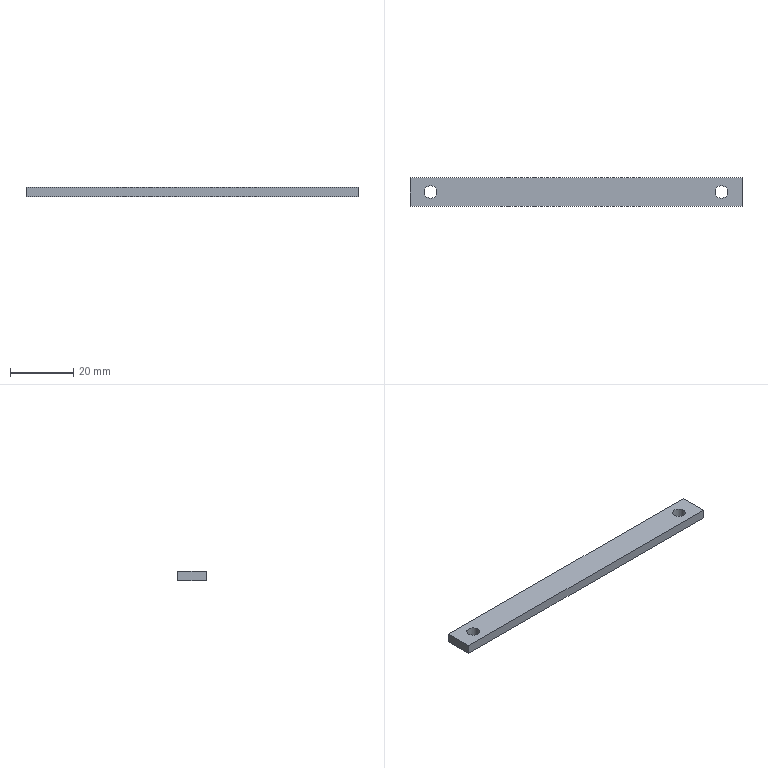Component | NX | GUIDE_PLATE_2 | 1 solid | 8 faces | box 105 x 9 x 3 mm | volume 2760 mm3 | plane 6 | cylinder 2 | commonest cylinder face diameters 4 x2
STEP:
#1=CARTESIAN_POINT('',(0.,0.,0.));
#2=DIRECTION('',(0.,0.,1.));
#3=DIRECTION('',(1.,0.,0.));
#4=AXIS2_PLACEMENT_3D('',#1,#2,#3);
#5=CARTESIAN_POINT('',(331.,-76.,115.5));
#6=VERTEX_POINT('',#5);
#7=CARTESIAN_POINT('',(226.,-76.,115.5));
#8=VERTEX_POINT('',#7);
#9=CARTESIAN_POINT('',(331.,-76.,115.5));
#10=DIRECTION('',(-1.,0.,0.));
#11=VECTOR('',#10,1.);
#12=LINE('',#9,#11);
#13=CARTESIAN_POINT('',(331.,-76.,118.5));
#14=DIRECTION('',(0.,-1.,0.));
#15=DIRECTION('',(0.,0.,-1.));
#16=AXIS2_PLACEMENT_3D('',#13,#14,#15);
#17=PLANE('',#16);
#18=CARTESIAN_POINT('',(3.,0.));
#19=DIRECTION('',(0.,-1.));
#20=VECTOR('',#19,1.);
#21=LINE('',#18,#20);
#22=(GEOMETRIC_REPRESENTATION_CONTEXT(2)PARAMETRIC_REPRESENTATION_CONTEXT()REPRESENTATION_CONTEXT('',''));
#23=DEFINITIONAL_REPRESENTATION('',(#21),#22);
#24=PCURVE('',#17,#23);
#25=CARTESIAN_POINT('',(324.5,-71.5,115.5));
#26=DIRECTION('',(0.,0.,1.));
#27=DIRECTION('',(1.,0.,0.));
#28=AXIS2_PLACEMENT_3D('',#25,#26,#27);
#29=PLANE('',#28);
#30=CARTESIAN_POINT('',(6.5,-4.5));
#31=DIRECTION('',(-1.,0.));
#32=VECTOR('',#31,1.);
#33=LINE('',#30,#32);
#34=(GEOMETRIC_REPRESENTATION_CONTEXT(2)PARAMETRIC_REPRESENTATION_CONTEXT()REPRESENTATION_CONTEXT('',''));
#35=DEFINITIONAL_REPRESENTATION('',(#33),#34);
#36=PCURVE('',#29,#35);
#37=SURFACE_CURVE('',#12,(#24,#36),.PCURVE_S1.);
#38=EDGE_CURVE('',#6,#8,#37,.T.);
#39=ORIENTED_EDGE('',*,*,#38,.F.);
#40=CARTESIAN_POINT('',(331.,-76.,118.5));
#41=VERTEX_POINT('',#40);
#42=CARTESIAN_POINT('',(331.,-76.,118.5));
#43=DIRECTION('',(0.,0.,-1.));
#44=VECTOR('',#43,1.);
#45=LINE('',#42,#44);
#46=CARTESIAN_POINT('',(0.,0.));
#47=DIRECTION('',(1.,0.));
#48=VECTOR('',#47,1.);
#49=LINE('',#46,#48);
#50=(GEOMETRIC_REPRESENTATION_CONTEXT(2)PARAMETRIC_REPRESENTATION_CONTEXT()REPRESENTATION_CONTEXT('',''));
#51=DEFINITIONAL_REPRESENTATION('',(#49),#50);
#52=PCURVE('',#17,#51);
#53=CARTESIAN_POINT('',(331.,-67.,118.5));
#54=DIRECTION('',(1.,0.,0.));
#55=DIRECTION('',(0.,0.,-1.));
#56=AXIS2_PLACEMENT_3D('',#53,#54,#55);
#57=PLANE('',#56);
#58=CARTESIAN_POINT('',(0.,-9.));
#59=DIRECTION('',(1.,0.));
#60=VECTOR('',#59,1.);
#61=LINE('',#58,#60);
#62=(GEOMETRIC_REPRESENTATION_CONTEXT(2)PARAMETRIC_REPRESENTATION_CONTEXT()REPRESENTATION_CONTEXT('',''));
#63=DEFINITIONAL_REPRESENTATION('',(#61),#62);
#64=PCURVE('',#57,#63);
#65=SURFACE_CURVE('',#45,(#52,#64),.PCURVE_S1.);
#66=EDGE_CURVE('',#41,#6,#65,.T.);
#67=ORIENTED_EDGE('',*,*,#66,.F.);
#68=CARTESIAN_POINT('',(226.,-76.,118.5));
#69=VERTEX_POINT('',#68);
#70=CARTESIAN_POINT('',(331.,-76.,118.5));
#71=DIRECTION('',(-1.,0.,0.));
#72=VECTOR('',#71,1.);
#73=LINE('',#70,#72);
#74=CARTESIAN_POINT('',(0.,0.));
#75=DIRECTION('',(0.,-1.));
#76=VECTOR('',#75,1.);
#77=LINE('',#74,#76);
#78=(GEOMETRIC_REPRESENTATION_CONTEXT(2)PARAMETRIC_REPRESENTATION_CONTEXT()REPRESENTATION_CONTEXT('',''));
#79=DEFINITIONAL_REPRESENTATION('',(#77),#78);
#80=PCURVE('',#17,#79);
#81=CARTESIAN_POINT('',(324.5,-71.5,118.5));
#82=DIRECTION('',(0.,0.,1.));
#83=DIRECTION('',(1.,0.,0.));
#84=AXIS2_PLACEMENT_3D('',#81,#82,#83);
#85=PLANE('',#84);
#86=CARTESIAN_POINT('',(6.5,-4.5));
#87=DIRECTION('',(-1.,0.));
#88=VECTOR('',#87,1.);
#89=LINE('',#86,#88);
#90=(GEOMETRIC_REPRESENTATION_CONTEXT(2)PARAMETRIC_REPRESENTATION_CONTEXT()REPRESENTATION_CONTEXT('',''));
#91=DEFINITIONAL_REPRESENTATION('',(#89),#90);
#92=PCURVE('',#85,#91);
#93=SURFACE_CURVE('',#73,(#80,#92),.PCURVE_S1.);
#94=EDGE_CURVE('',#41,#69,#93,.T.);
#95=ORIENTED_EDGE('',*,*,#94,.T.);
#96=CARTESIAN_POINT('',(226.,-76.,118.5));
#97=DIRECTION('',(0.,0.,-1.));
#98=VECTOR('',#97,1.);
#99=LINE('',#96,#98);
#100=CARTESIAN_POINT('',(0.,-105.));
#101=DIRECTION('',(1.,0.));
#102=VECTOR('',#101,1.);
#103=LINE('',#100,#102);
#104=(GEOMETRIC_REPRESENTATION_CONTEXT(2)PARAMETRIC_REPRESENTATION_CONTEXT()REPRESENTATION_CONTEXT('',''));
#105=DEFINITIONAL_REPRESENTATION('',(#103),#104);
#106=PCURVE('',#17,#105);
#107=CARTESIAN_POINT('',(226.,-76.,118.5));
#108=DIRECTION('',(-1.,0.,0.));
#109=DIRECTION('',(0.,0.,1.));
#110=AXIS2_PLACEMENT_3D('',#107,#108,#109);
#111=PLANE('',#110);
#112=CARTESIAN_POINT('',(0.,0.));
#113=DIRECTION('',(-1.,0.));
#114=VECTOR('',#113,1.);
#115=LINE('',#112,#114);
#116=(GEOMETRIC_REPRESENTATION_CONTEXT(2)PARAMETRIC_REPRESENTATION_CONTEXT()REPRESENTATION_CONTEXT('',''));
#117=DEFINITIONAL_REPRESENTATION('',(#115),#116);
#118=PCURVE('',#111,#117);
#119=SURFACE_CURVE('',#99,(#106,#118),.PCURVE_S1.);
#120=EDGE_CURVE('',#69,#8,#119,.T.);
#121=ORIENTED_EDGE('',*,*,#120,.T.);
#122=EDGE_LOOP('',(#39,#67,#95,#121));
#123=FACE_BOUND('',#122,.T.);
#124=ADVANCED_FACE('',(#123),#17,.T.);
#125=CARTESIAN_POINT('',(226.,-67.,115.5));
#126=VERTEX_POINT('',#125);
#127=CARTESIAN_POINT('',(226.,-76.,115.5));
#128=DIRECTION('',(0.,1.,0.));
#129=VECTOR('',#128,1.);
#130=LINE('',#127,#129);
#131=CARTESIAN_POINT('',(-3.,0.));
#132=DIRECTION('',(0.,1.));
#133=VECTOR('',#132,1.);
#134=LINE('',#131,#133);
#135=(GEOMETRIC_REPRESENTATION_CONTEXT(2)PARAMETRIC_REPRESENTATION_CONTEXT()REPRESENTATION_CONTEXT('',''));
#136=DEFINITIONAL_REPRESENTATION('',(#134),#135);
#137=PCURVE('',#111,#136);
#138=CARTESIAN_POINT('',(-98.5,-4.5));
#139=DIRECTION('',(0.,1.));
#140=VECTOR('',#139,1.);
#141=LINE('',#138,#140);
#142=(GEOMETRIC_REPRESENTATION_CONTEXT(2)PARAMETRIC_REPRESENTATION_CONTEXT()REPRESENTATION_CONTEXT('',''));
#143=DEFINITIONAL_REPRESENTATION('',(#141),#142);
#144=PCURVE('',#29,#143);
#145=SURFACE_CURVE('',#130,(#137,#144),.PCURVE_S1.);
#146=EDGE_CURVE('',#8,#126,#145,.T.);
#147=ORIENTED_EDGE('',*,*,#146,.F.);
#148=ORIENTED_EDGE('',*,*,#120,.F.);
#149=CARTESIAN_POINT('',(226.,-67.,118.5));
#150=VERTEX_POINT('',#149);
#151=CARTESIAN_POINT('',(226.,-76.,118.5));
#152=DIRECTION('',(0.,1.,0.));
#153=VECTOR('',#152,1.);
#154=LINE('',#151,#153);
#155=CARTESIAN_POINT('',(0.,0.));
#156=DIRECTION('',(0.,1.));
#157=VECTOR('',#156,1.);
#158=LINE('',#155,#157);
#159=(GEOMETRIC_REPRESENTATION_CONTEXT(2)PARAMETRIC_REPRESENTATION_CONTEXT()REPRESENTATION_CONTEXT('',''));
#160=DEFINITIONAL_REPRESENTATION('',(#158),#159);
#161=PCURVE('',#111,#160);
#162=CARTESIAN_POINT('',(-98.5,-4.5));
#163=DIRECTION('',(0.,1.));
#164=VECTOR('',#163,1.);
#165=LINE('',#162,#164);
#166=(GEOMETRIC_REPRESENTATION_CONTEXT(2)PARAMETRIC_REPRESENTATION_CONTEXT()REPRESENTATION_CONTEXT('',''));
#167=DEFINITIONAL_REPRESENTATION('',(#165),#166);
#168=PCURVE('',#85,#167);
#169=SURFACE_CURVE('',#154,(#161,#168),.PCURVE_S1.);
#170=EDGE_CURVE('',#69,#150,#169,.T.);
#171=ORIENTED_EDGE('',*,*,#170,.T.);
#172=CARTESIAN_POINT('',(226.,-67.,118.5));
#173=DIRECTION('',(0.,0.,-1.));
#174=VECTOR('',#173,1.);
#175=LINE('',#172,#174);
#176=CARTESIAN_POINT('',(0.,9.));
#177=DIRECTION('',(-1.,0.));
#178=VECTOR('',#177,1.);
#179=LINE('',#176,#178);
#180=(GEOMETRIC_REPRESENTATION_CONTEXT(2)PARAMETRIC_REPRESENTATION_CONTEXT()REPRESENTATION_CONTEXT('',''));
#181=DEFINITIONAL_REPRESENTATION('',(#179),#180);
#182=PCURVE('',#111,#181);
#183=CARTESIAN_POINT('',(226.,-67.,118.5));
#184=DIRECTION('',(0.,1.,0.));
#185=DIRECTION('',(0.,0.,1.));
#186=AXIS2_PLACEMENT_3D('',#183,#184,#185);
#187=PLANE('',#186);
#188=CARTESIAN_POINT('',(0.,0.));
#189=DIRECTION('',(-1.,0.));
#190=VECTOR('',#189,1.);
#191=LINE('',#188,#190);
#192=(GEOMETRIC_REPRESENTATION_CONTEXT(2)PARAMETRIC_REPRESENTATION_CONTEXT()REPRESENTATION_CONTEXT('',''));
#193=DEFINITIONAL_REPRESENTATION('',(#191),#192);
#194=PCURVE('',#187,#193);
#195=SURFACE_CURVE('',#175,(#182,#194),.PCURVE_S1.);
#196=EDGE_CURVE('',#150,#126,#195,.T.);
#197=ORIENTED_EDGE('',*,*,#196,.T.);
#198=EDGE_LOOP('',(#147,#148,#171,#197));
#199=FACE_BOUND('',#198,.T.);
#200=ADVANCED_FACE('',(#199),#111,.T.);
#201=CARTESIAN_POINT('',(331.,-67.,115.5));
#202=VERTEX_POINT('',#201);
#203=CARTESIAN_POINT('',(226.,-67.,115.5));
#204=DIRECTION('',(1.,0.,0.));
#205=VECTOR('',#204,1.);
#206=LINE('',#203,#205);
#207=CARTESIAN_POINT('',(-3.,0.));
#208=DIRECTION('',(0.,1.));
#209=VECTOR('',#208,1.);
#210=LINE('',#207,#209);
#211=(GEOMETRIC_REPRESENTATION_CONTEXT(2)PARAMETRIC_REPRESENTATION_CONTEXT()REPRESENTATION_CONTEXT('',''));
#212=DEFINITIONAL_REPRESENTATION('',(#210),#211);
#213=PCURVE('',#187,#212);
#214=CARTESIAN_POINT('',(-98.5,4.5));
#215=DIRECTION('',(1.,0.));
#216=VECTOR('',#215,1.);
#217=LINE('',#214,#216);
#218=(GEOMETRIC_REPRESENTATION_CONTEXT(2)PARAMETRIC_REPRESENTATION_CONTEXT()REPRESENTATION_CONTEXT('',''));
#219=DEFINITIONAL_REPRESENTATION('',(#217),#218);
#220=PCURVE('',#29,#219);
#221=SURFACE_CURVE('',#206,(#213,#220),.PCURVE_S1.);
#222=EDGE_CURVE('',#126,#202,#221,.T.);
#223=ORIENTED_EDGE('',*,*,#222,.F.);
#224=ORIENTED_EDGE('',*,*,#196,.F.);
#225=CARTESIAN_POINT('',(331.,-67.,118.5));
#226=VERTEX_POINT('',#225);
#227=CARTESIAN_POINT('',(226.,-67.,118.5));
#228=DIRECTION('',(1.,0.,0.));
#229=VECTOR('',#228,1.);
#230=LINE('',#227,#229);
#231=CARTESIAN_POINT('',(0.,0.));
#232=DIRECTION('',(0.,1.));
#233=VECTOR('',#232,1.);
#234=LINE('',#231,#233);
#235=(GEOMETRIC_REPRESENTATION_CONTEXT(2)PARAMETRIC_REPRESENTATION_CONTEXT()REPRESENTATION_CONTEXT('',''));
#236=DEFINITIONAL_REPRESENTATION('',(#234),#235);
#237=PCURVE('',#187,#236);
#238=CARTESIAN_POINT('',(-98.5,4.5));
#239=DIRECTION('',(1.,0.));
#240=VECTOR('',#239,1.);
#241=LINE('',#238,#240);
#242=(GEOMETRIC_REPRESENTATION_CONTEXT(2)PARAMETRIC_REPRESENTATION_CONTEXT()REPRESENTATION_CONTEXT('',''));
#243=DEFINITIONAL_REPRESENTATION('',(#241),#242);
#244=PCURVE('',#85,#243);
#245=SURFACE_CURVE('',#230,(#237,#244),.PCURVE_S1.);
#246=EDGE_CURVE('',#150,#226,#245,.T.);
#247=ORIENTED_EDGE('',*,*,#246,.T.);
#248=CARTESIAN_POINT('',(331.,-67.,118.5));
#249=DIRECTION('',(0.,0.,-1.));
#250=VECTOR('',#249,1.);
#251=LINE('',#248,#250);
#252=CARTESIAN_POINT('',(0.,105.));
#253=DIRECTION('',(-1.,0.));
#254=VECTOR('',#253,1.);
#255=LINE('',#252,#254);
#256=(GEOMETRIC_REPRESENTATION_CONTEXT(2)PARAMETRIC_REPRESENTATION_CONTEXT()REPRESENTATION_CONTEXT('',''));
#257=DEFINITIONAL_REPRESENTATION('',(#255),#256);
#258=PCURVE('',#187,#257);
#259=CARTESIAN_POINT('',(0.,0.));
#260=DIRECTION('',(1.,0.));
#261=VECTOR('',#260,1.);
#262=LINE('',#259,#261);
#263=(GEOMETRIC_REPRESENTATION_CONTEXT(2)PARAMETRIC_REPRESENTATION_CONTEXT()REPRESENTATION_CONTEXT('',''));
#264=DEFINITIONAL_REPRESENTATION('',(#262),#263);
#265=PCURVE('',#57,#264);
#266=SURFACE_CURVE('',#251,(#258,#265),.PCURVE_S1.);
#267=EDGE_CURVE('',#226,#202,#266,.T.);
#268=ORIENTED_EDGE('',*,*,#267,.T.);
#269=EDGE_LOOP('',(#223,#224,#247,#268));
#270=FACE_BOUND('',#269,.T.);
#271=ADVANCED_FACE('',(#270),#187,.T.);
#272=CARTESIAN_POINT('',(322.5,-71.5,118.5));
#273=VERTEX_POINT('',#272);
#274=CARTESIAN_POINT('',(324.5,-71.5,118.5));
#275=DIRECTION('',(0.,0.,1.));
#276=DIRECTION('',(-1.,0.,0.));
#277=AXIS2_PLACEMENT_3D('',#274,#275,#276);
#278=CIRCLE('',#277,2.);
#279=CARTESIAN_POINT('',(324.5,-71.5,118.5));
#280=DIRECTION('',(0.,0.,-1.));
#281=DIRECTION('',(-1.,0.,0.));
#282=AXIS2_PLACEMENT_3D('',#279,#280,#281);
#283=CYLINDRICAL_SURFACE('',#282,2.);
#284=CARTESIAN_POINT('',(6.283,0.));
#285=DIRECTION('',(-1.,0.));
#286=VECTOR('',#285,1.);
#287=LINE('',#284,#286);
#288=(GEOMETRIC_REPRESENTATION_CONTEXT(2)PARAMETRIC_REPRESENTATION_CONTEXT()REPRESENTATION_CONTEXT('',''));
#289=DEFINITIONAL_REPRESENTATION('',(#287),#288);
#290=PCURVE('',#283,#289);
#291=CARTESIAN_POINT('',(0.,0.));
#292=DIRECTION('',(-1.,0.));
#293=AXIS2_PLACEMENT_2D('',#291,#292);
#294=CIRCLE('',#293,2.);
#295=(GEOMETRIC_REPRESENTATION_CONTEXT(2)PARAMETRIC_REPRESENTATION_CONTEXT()REPRESENTATION_CONTEXT('',''));
#296=DEFINITIONAL_REPRESENTATION('',(#294),#295);
#297=PCURVE('',#85,#296);
#298=SURFACE_CURVE('',#278,(#290,#297),.PCURVE_S1.);
#299=EDGE_CURVE('',#273,#273,#298,.T.);
#300=ORIENTED_EDGE('',*,*,#299,.F.);
#301=CARTESIAN_POINT('',(322.5,-71.5,115.5));
#302=VERTEX_POINT('',#301);
#303=CARTESIAN_POINT('',(322.5,-71.5,118.5));
#304=CARTESIAN_POINT('',(322.5,-71.5,115.5));
#305=B_SPLINE_CURVE_WITH_KNOTS('',1,(#303,#304),.UNSPECIFIED.,.F.,.F.,(2,2),(0.,3.),.PIECEWISE_BEZIER_KNOTS.);
#306=CARTESIAN_POINT('',(6.283,0.));
#307=DIRECTION('',(0.,1.));
#308=VECTOR('',#307,1.);
#309=LINE('',#306,#308);
#310=(GEOMETRIC_REPRESENTATION_CONTEXT(2)PARAMETRIC_REPRESENTATION_CONTEXT()REPRESENTATION_CONTEXT('',''));
#311=DEFINITIONAL_REPRESENTATION('',(#309),#310);
#312=PCURVE('',#283,#311);
#313=CARTESIAN_POINT('',(0.,0.));
#314=DIRECTION('',(0.,1.));
#315=VECTOR('',#314,1.);
#316=LINE('',#313,#315);
#317=(GEOMETRIC_REPRESENTATION_CONTEXT(2)PARAMETRIC_REPRESENTATION_CONTEXT()REPRESENTATION_CONTEXT('',''));
#318=DEFINITIONAL_REPRESENTATION('',(#316),#317);
#319=PCURVE('',#283,#318);
#320=SEAM_CURVE('',#305,(#312,#319),.PCURVE_S1.);
#321=EDGE_CURVE('',#273,#302,#320,.T.);
#322=ORIENTED_EDGE('',*,*,#321,.T.);
#323=CARTESIAN_POINT('',(324.5,-71.5,115.5));
#324=DIRECTION('',(0.,0.,1.));
#325=DIRECTION('',(-1.,0.,0.));
#326=AXIS2_PLACEMENT_3D('',#323,#324,#325);
#327=CIRCLE('',#326,2.);
#328=CARTESIAN_POINT('',(6.283,3.));
#329=DIRECTION('',(-1.,0.));
#330=VECTOR('',#329,1.);
#331=LINE('',#328,#330);
#332=(GEOMETRIC_REPRESENTATION_CONTEXT(2)PARAMETRIC_REPRESENTATION_CONTEXT()REPRESENTATION_CONTEXT('',''));
#333=DEFINITIONAL_REPRESENTATION('',(#331),#332);
#334=PCURVE('',#283,#333);
#335=CARTESIAN_POINT('',(0.,0.));
#336=DIRECTION('',(-1.,0.));
#337=AXIS2_PLACEMENT_2D('',#335,#336);
#338=CIRCLE('',#337,2.);
#339=(GEOMETRIC_REPRESENTATION_CONTEXT(2)PARAMETRIC_REPRESENTATION_CONTEXT()REPRESENTATION_CONTEXT('',''));
#340=DEFINITIONAL_REPRESENTATION('',(#338),#339);
#341=PCURVE('',#29,#340);
#342=SURFACE_CURVE('',#327,(#334,#341),.PCURVE_S1.);
#343=EDGE_CURVE('',#302,#302,#342,.T.);
#344=ORIENTED_EDGE('',*,*,#343,.T.);
#345=ORIENTED_EDGE('',*,*,#321,.F.);
#346=EDGE_LOOP('',(#300,#322,#344,#345));
#347=FACE_BOUND('',#346,.F.);
#348=ADVANCED_FACE('',(#347),#283,.F.);
#349=CARTESIAN_POINT('',(331.,-67.,115.5));
#350=DIRECTION('',(0.,-1.,0.));
#351=VECTOR('',#350,1.);
#352=LINE('',#349,#351);
#353=CARTESIAN_POINT('',(3.,0.));
#354=DIRECTION('',(0.,-1.));
#355=VECTOR('',#354,1.);
#356=LINE('',#353,#355);
#357=(GEOMETRIC_REPRESENTATION_CONTEXT(2)PARAMETRIC_REPRESENTATION_CONTEXT()REPRESENTATION_CONTEXT('',''));
#358=DEFINITIONAL_REPRESENTATION('',(#356),#357);
#359=PCURVE('',#57,#358);
#360=CARTESIAN_POINT('',(6.5,4.5));
#361=DIRECTION('',(0.,-1.));
#362=VECTOR('',#361,1.);
#363=LINE('',#360,#362);
#364=(GEOMETRIC_REPRESENTATION_CONTEXT(2)PARAMETRIC_REPRESENTATION_CONTEXT()REPRESENTATION_CONTEXT('',''));
#365=DEFINITIONAL_REPRESENTATION('',(#363),#364);
#366=PCURVE('',#29,#365);
#367=SURFACE_CURVE('',#352,(#359,#366),.PCURVE_S1.);
#368=EDGE_CURVE('',#202,#6,#367,.T.);
#369=ORIENTED_EDGE('',*,*,#368,.F.);
#370=ORIENTED_EDGE('',*,*,#267,.F.);
#371=CARTESIAN_POINT('',(331.,-67.,118.5));
#372=DIRECTION('',(0.,-1.,0.));
#373=VECTOR('',#372,1.);
#374=LINE('',#371,#373);
#375=CARTESIAN_POINT('',(0.,0.));
#376=DIRECTION('',(0.,-1.));
#377=VECTOR('',#376,1.);
#378=LINE('',#375,#377);
#379=(GEOMETRIC_REPRESENTATION_CONTEXT(2)PARAMETRIC_REPRESENTATION_CONTEXT()REPRESENTATION_CONTEXT('',''));
#380=DEFINITIONAL_REPRESENTATION('',(#378),#379);
#381=PCURVE('',#57,#380);
#382=CARTESIAN_POINT('',(6.5,4.5));
#383=DIRECTION('',(0.,-1.));
#384=VECTOR('',#383,1.);
#385=LINE('',#382,#384);
#386=(GEOMETRIC_REPRESENTATION_CONTEXT(2)PARAMETRIC_REPRESENTATION_CONTEXT()REPRESENTATION_CONTEXT('',''));
#387=DEFINITIONAL_REPRESENTATION('',(#385),#386);
#388=PCURVE('',#85,#387);
#389=SURFACE_CURVE('',#374,(#381,#388),.PCURVE_S1.);
#390=EDGE_CURVE('',#226,#41,#389,.T.);
#391=ORIENTED_EDGE('',*,*,#390,.T.);
#392=ORIENTED_EDGE('',*,*,#66,.T.);
#393=EDGE_LOOP('',(#369,#370,#391,#392));
#394=FACE_BOUND('',#393,.T.);
#395=ADVANCED_FACE('',(#394),#57,.T.);
#396=CARTESIAN_POINT('',(234.5,-71.5,118.5));
#397=VERTEX_POINT('',#396);
#398=CARTESIAN_POINT('',(232.5,-71.5,118.5));
#399=DIRECTION('',(0.,0.,-1.));
#400=DIRECTION('',(1.,0.,0.));
#401=AXIS2_PLACEMENT_3D('',#398,#399,#400);
#402=CIRCLE('',#401,2.);
#403=CARTESIAN_POINT('',(232.5,-71.5,118.5));
#404=DIRECTION('',(0.,0.,-1.));
#405=DIRECTION('',(-1.,0.,0.));
#406=AXIS2_PLACEMENT_3D('',#403,#404,#405);
#407=CYLINDRICAL_SURFACE('',#406,2.);
#408=CARTESIAN_POINT('',(3.142,0.));
#409=DIRECTION('',(1.,0.));
#410=VECTOR('',#409,1.);
#411=LINE('',#408,#410);
#412=(GEOMETRIC_REPRESENTATION_CONTEXT(2)PARAMETRIC_REPRESENTATION_CONTEXT()REPRESENTATION_CONTEXT('',''));
#413=DEFINITIONAL_REPRESENTATION('',(#411),#412);
#414=PCURVE('',#407,#413);
#415=CARTESIAN_POINT('',(-90.,0.));
#416=CARTESIAN_POINT('',(-90.,-3.464));
#417=CARTESIAN_POINT('',(-93.,-1.732));
#418=CARTESIAN_POINT('',(-96.,-0.));
#419=CARTESIAN_POINT('',(-93.,1.732));
#420=CARTESIAN_POINT('',(-90.,3.464));
#421=CARTESIAN_POINT('',(-90.,0.));
#422=(BOUNDED_CURVE()B_SPLINE_CURVE(2,(#415,#416,#417,#418,#419,#420,#421),.UNSPECIFIED.,.T.,.F.)B_SPLINE_CURVE_WITH_KNOTS((1,2,2,2,2,1),(-2.094,0.,2.094,4.189,6.283,8.378),.UNSPECIFIED.)CURVE()GEOMETRIC_REPRESENTATION_ITEM()RATIONAL_B_SPLINE_CURVE((1.,0.5,1.,0.5,1.,0.5,1.))REPRESENTATION_ITEM(''));
#423=(GEOMETRIC_REPRESENTATION_CONTEXT(2)PARAMETRIC_REPRESENTATION_CONTEXT()REPRESENTATION_CONTEXT('',''));
#424=DEFINITIONAL_REPRESENTATION('',(#422),#423);
#425=PCURVE('',#85,#424);
#426=SURFACE_CURVE('',#402,(#414,#425),.PCURVE_S1.);
#427=EDGE_CURVE('',#397,#397,#426,.T.);
#428=ORIENTED_EDGE('',*,*,#427,.T.);
#429=CARTESIAN_POINT('',(234.5,-71.5,115.5));
#430=VERTEX_POINT('',#429);
#431=CARTESIAN_POINT('',(234.5,-71.5,118.5));
#432=CARTESIAN_POINT('',(234.5,-71.5,115.5));
#433=B_SPLINE_CURVE_WITH_KNOTS('',1,(#431,#432),.UNSPECIFIED.,.F.,.F.,(2,2),(0.,3.),.PIECEWISE_BEZIER_KNOTS.);
#434=CARTESIAN_POINT('',(9.425,0.));
#435=DIRECTION('',(0.,1.));
#436=VECTOR('',#435,1.);
#437=LINE('',#434,#436);
#438=(GEOMETRIC_REPRESENTATION_CONTEXT(2)PARAMETRIC_REPRESENTATION_CONTEXT()REPRESENTATION_CONTEXT('',''));
#439=DEFINITIONAL_REPRESENTATION('',(#437),#438);
#440=PCURVE('',#407,#439);
#441=CARTESIAN_POINT('',(3.142,0.));
#442=DIRECTION('',(0.,1.));
#443=VECTOR('',#442,1.);
#444=LINE('',#441,#443);
#445=(GEOMETRIC_REPRESENTATION_CONTEXT(2)PARAMETRIC_REPRESENTATION_CONTEXT()REPRESENTATION_CONTEXT('',''));
#446=DEFINITIONAL_REPRESENTATION('',(#444),#445);
#447=PCURVE('',#407,#446);
#448=SEAM_CURVE('',#433,(#440,#447),.PCURVE_S1.);
#449=EDGE_CURVE('',#397,#430,#448,.T.);
#450=ORIENTED_EDGE('',*,*,#449,.T.);
#451=CARTESIAN_POINT('',(232.5,-71.5,115.5));
#452=DIRECTION('',(0.,0.,-1.));
#453=DIRECTION('',(1.,0.,0.));
#454=AXIS2_PLACEMENT_3D('',#451,#452,#453);
#455=CIRCLE('',#454,2.);
#456=CARTESIAN_POINT('',(3.142,3.));
#457=DIRECTION('',(1.,0.));
#458=VECTOR('',#457,1.);
#459=LINE('',#456,#458);
#460=(GEOMETRIC_REPRESENTATION_CONTEXT(2)PARAMETRIC_REPRESENTATION_CONTEXT()REPRESENTATION_CONTEXT('',''));
#461=DEFINITIONAL_REPRESENTATION('',(#459),#460);
#462=PCURVE('',#407,#461);
#463=CARTESIAN_POINT('',(-90.,0.));
#464=CARTESIAN_POINT('',(-90.,-3.464));
#465=CARTESIAN_POINT('',(-93.,-1.732));
#466=CARTESIAN_POINT('',(-96.,-0.));
#467=CARTESIAN_POINT('',(-93.,1.732));
#468=CARTESIAN_POINT('',(-90.,3.464));
#469=CARTESIAN_POINT('',(-90.,0.));
#470=(BOUNDED_CURVE()B_SPLINE_CURVE(2,(#463,#464,#465,#466,#467,#468,#469),.UNSPECIFIED.,.T.,.F.)B_SPLINE_CURVE_WITH_KNOTS((1,2,2,2,2,1),(-2.094,0.,2.094,4.189,6.283,8.378),.UNSPECIFIED.)CURVE()GEOMETRIC_REPRESENTATION_ITEM()RATIONAL_B_SPLINE_CURVE((1.,0.5,1.,0.5,1.,0.5,1.))REPRESENTATION_ITEM(''));
#471=(GEOMETRIC_REPRESENTATION_CONTEXT(2)PARAMETRIC_REPRESENTATION_CONTEXT()REPRESENTATION_CONTEXT('',''));
#472=DEFINITIONAL_REPRESENTATION('',(#470),#471);
#473=PCURVE('',#29,#472);
#474=SURFACE_CURVE('',#455,(#462,#473),.PCURVE_S1.);
#475=EDGE_CURVE('',#430,#430,#474,.T.);
#476=ORIENTED_EDGE('',*,*,#475,.F.);
#477=ORIENTED_EDGE('',*,*,#449,.F.);
#478=EDGE_LOOP('',(#428,#450,#476,#477));
#479=FACE_BOUND('',#478,.F.);
#480=ADVANCED_FACE('',(#479),#407,.F.);
#481=ORIENTED_EDGE('',*,*,#94,.F.);
#482=ORIENTED_EDGE('',*,*,#390,.F.);
#483=ORIENTED_EDGE('',*,*,#246,.F.);
#484=ORIENTED_EDGE('',*,*,#170,.F.);
#485=EDGE_LOOP('',(#481,#482,#483,#484));
#486=FACE_BOUND('',#485,.T.);
#487=ORIENTED_EDGE('',*,*,#299,.F.);
#488=EDGE_LOOP('',(#487));
#489=FACE_BOUND('',#488,.T.);
#490=ORIENTED_EDGE('',*,*,#427,.T.);
#491=EDGE_LOOP('',(#490));
#492=FACE_BOUND('',#491,.T.);
#493=ADVANCED_FACE('',(#486,#489,#492),#85,.T.);
#494=ORIENTED_EDGE('',*,*,#38,.T.);
#495=ORIENTED_EDGE('',*,*,#146,.T.);
#496=ORIENTED_EDGE('',*,*,#222,.T.);
#497=ORIENTED_EDGE('',*,*,#368,.T.);
#498=EDGE_LOOP('',(#494,#495,#496,#497));
#499=FACE_BOUND('',#498,.T.);
#500=ORIENTED_EDGE('',*,*,#343,.T.);
#501=EDGE_LOOP('',(#500));
#502=FACE_BOUND('',#501,.T.);
#503=ORIENTED_EDGE('',*,*,#475,.F.);
#504=EDGE_LOOP('',(#503));
#505=FACE_BOUND('',#504,.T.);
#506=ADVANCED_FACE('',(#499,#502,#505),#29,.F.);
#507=CLOSED_SHELL('',(#124,#200,#271,#348,#395,#480,#493,#506));
#508=MANIFOLD_SOLID_BREP('',#507);
#509=(LENGTH_UNIT()NAMED_UNIT(*)SI_UNIT(.MILLI.,.METRE.));
#510=UNCERTAINTY_MEASURE_WITH_UNIT(LENGTH_MEASURE(0.000002),#509,'','');
#511=(NAMED_UNIT(*)PLANE_ANGLE_UNIT()SI_UNIT($,.RADIAN.));
#512=(NAMED_UNIT(*)SI_UNIT($,.STERADIAN.)SOLID_ANGLE_UNIT());
#513=(GEOMETRIC_REPRESENTATION_CONTEXT(3)GLOBAL_UNCERTAINTY_ASSIGNED_CONTEXT((#510))GLOBAL_UNIT_ASSIGNED_CONTEXT((#509,#511,#512))REPRESENTATION_CONTEXT('',''));
#514=ADVANCED_BREP_SHAPE_REPRESENTATION('',(#4,#508),#513);